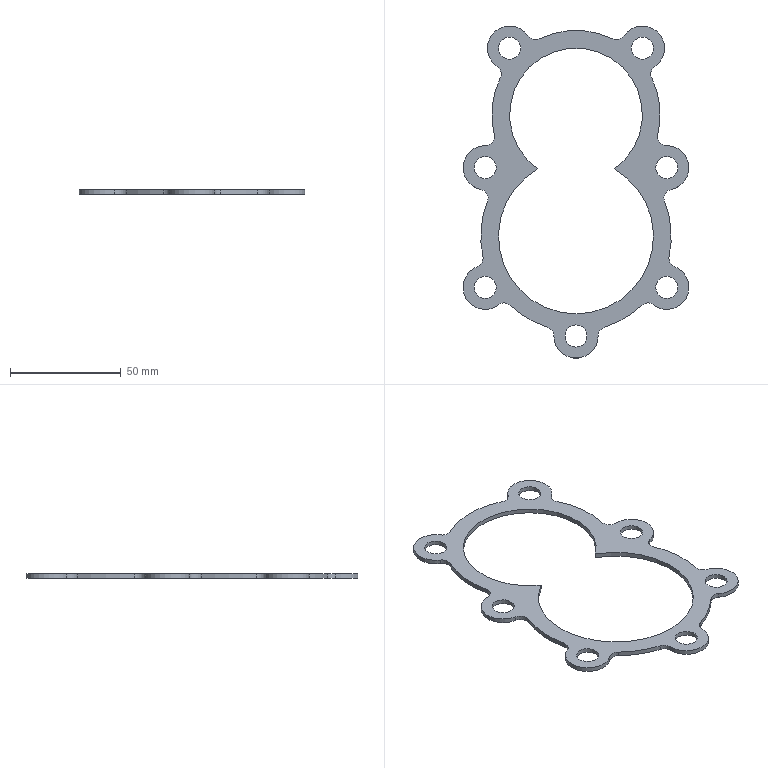Component | NX | 5_GASKET | 1 solid | 39 faces | volume 8295 mm3 | cylinder 37 | plane 2 | commonest cylinder face diameters 8 x14 20 x7 10 x7 86 x4 76 x3 70 x1 60 x1